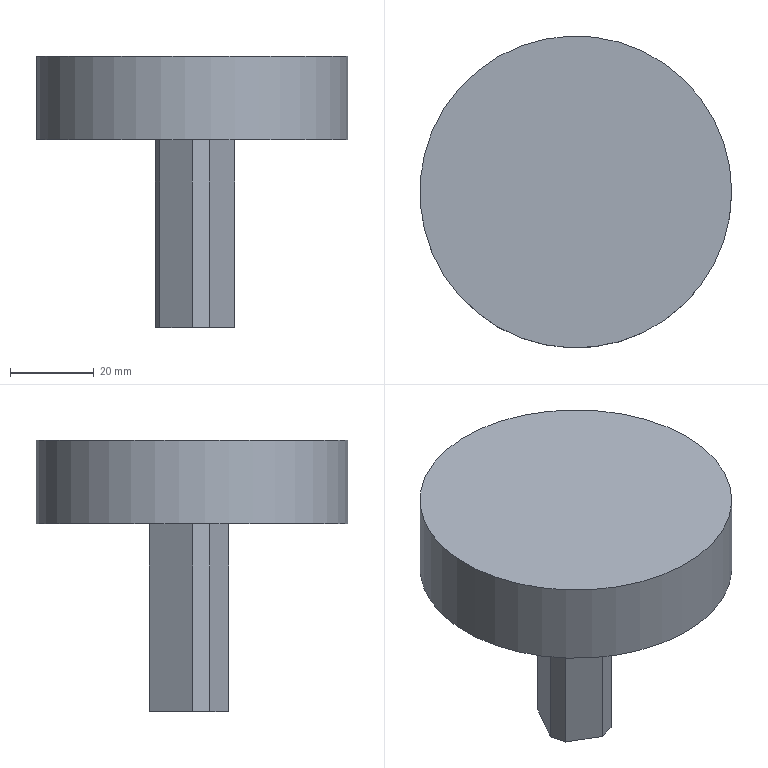Component | NX | CONNECTING_ROD | 1 solid | 17 faces | box 74.65 x 74.65 x 65 mm | volume 61981 mm3 | plane 12 | cylinder 4 | cone 1 | commonest cylinder face diameters 74.65 x1 66.65 x1 38.65 x1 8 x1
STEP:
#1=CARTESIAN_POINT('',(0.,0.,0.));
#2=DIRECTION('',(0.,0.,1.));
#3=DIRECTION('',(1.,0.,0.));
#4=AXIS2_PLACEMENT_3D('',#1,#2,#3);
#5=CARTESIAN_POINT('',(-5.912,-1.741,-7.5));
#6=VERTEX_POINT('',#5);
#7=CARTESIAN_POINT('',(3.75,14.995,-7.5));
#8=DIRECTION('',(0.,0.,-1.));
#9=DIRECTION('',(-0.5,-0.866,0.));
#10=AXIS2_PLACEMENT_3D('',#7,#8,#9);
#11=CIRCLE('',#10,19.325);
#12=CARTESIAN_POINT('',(3.75,14.995,-7.5));
#13=DIRECTION('',(0.,0.,-1.));
#14=DIRECTION('',(-0.5,-0.866,0.));
#15=AXIS2_PLACEMENT_3D('',#12,#13,#14);
#16=PLANE('',#15);
#17=CARTESIAN_POINT('',(0.,0.));
#18=DIRECTION('',(1.,0.));
#19=AXIS2_PLACEMENT_2D('',#17,#18);
#20=CIRCLE('',#19,19.325);
#21=(GEOMETRIC_REPRESENTATION_CONTEXT(2)PARAMETRIC_REPRESENTATION_CONTEXT()REPRESENTATION_CONTEXT('',''));
#22=DEFINITIONAL_REPRESENTATION('',(#20),#21);
#23=PCURVE('',#16,#22);
#24=CARTESIAN_POINT('',(3.75,14.995,7.5));
#25=DIRECTION('',(0.,0.,-1.));
#26=DIRECTION('',(-0.5,-0.866,0.));
#27=AXIS2_PLACEMENT_3D('',#24,#25,#26);
#28=CYLINDRICAL_SURFACE('',#27,19.325);
#29=CARTESIAN_POINT('',(0.,15.));
#30=DIRECTION('',(1.,0.));
#31=VECTOR('',#30,1.);
#32=LINE('',#29,#31);
#33=(GEOMETRIC_REPRESENTATION_CONTEXT(2)PARAMETRIC_REPRESENTATION_CONTEXT()REPRESENTATION_CONTEXT('',''));
#34=DEFINITIONAL_REPRESENTATION('',(#32),#33);
#35=PCURVE('',#28,#34);
#36=SURFACE_CURVE('',#11,(#23,#35),.PCURVE_S1.);
#37=EDGE_CURVE('',#6,#6,#36,.T.);
#38=ORIENTED_EDGE('',*,*,#37,.T.);
#39=EDGE_LOOP('',(#38));
#40=FACE_BOUND('',#39,.T.);
#41=CARTESIAN_POINT('',(1.005,25.24,-7.5));
#42=VERTEX_POINT('',#41);
#43=CARTESIAN_POINT('',(-4.995,14.848,-7.5));
#44=VERTEX_POINT('',#43);
#45=CARTESIAN_POINT('',(1.005,25.24,-7.5));
#46=DIRECTION('',(-0.5,-0.866,0.));
#47=VECTOR('',#46,1.);
#48=LINE('',#45,#47);
#49=CARTESIAN_POINT('',(-7.5,7.5));
#50=DIRECTION('',(1.,0.));
#51=VECTOR('',#50,1.);
#52=LINE('',#49,#51);
#53=(GEOMETRIC_REPRESENTATION_CONTEXT(2)PARAMETRIC_REPRESENTATION_CONTEXT()REPRESENTATION_CONTEXT('',''));
#54=DEFINITIONAL_REPRESENTATION('',(#52),#53);
#55=PCURVE('',#16,#54);
#56=CARTESIAN_POINT('',(1.005,25.24,-52.5));
#57=DIRECTION('',(-0.866,0.5,0.));
#58=DIRECTION('',(0.,0.,-1.));
#59=AXIS2_PLACEMENT_3D('',#56,#57,#58);
#60=PLANE('',#59);
#61=CARTESIAN_POINT('',(-45.,0.));
#62=DIRECTION('',(0.,1.));
#63=VECTOR('',#62,1.);
#64=LINE('',#61,#63);
#65=(GEOMETRIC_REPRESENTATION_CONTEXT(2)PARAMETRIC_REPRESENTATION_CONTEXT()REPRESENTATION_CONTEXT('',''));
#66=DEFINITIONAL_REPRESENTATION('',(#64),#65);
#67=PCURVE('',#60,#66);
#68=SURFACE_CURVE('',#48,(#55,#67),.PCURVE_S1.);
#69=EDGE_CURVE('',#42,#44,#68,.T.);
#70=ORIENTED_EDGE('',*,*,#69,.T.);
#71=CARTESIAN_POINT('',(-3.897,10.75,-7.5));
#72=VERTEX_POINT('',#71);
#73=CARTESIAN_POINT('',(-4.995,14.848,-7.5));
#74=DIRECTION('',(0.2588,-0.9659,0.));
#75=VECTOR('',#74,1.);
#76=LINE('',#73,#75);
#77=CARTESIAN_POINT('',(4.5,7.5));
#78=DIRECTION('',(0.7071,-0.7071));
#79=VECTOR('',#78,1.);
#80=LINE('',#77,#79);
#81=(GEOMETRIC_REPRESENTATION_CONTEXT(2)PARAMETRIC_REPRESENTATION_CONTEXT()REPRESENTATION_CONTEXT('',''));
#82=DEFINITIONAL_REPRESENTATION('',(#80),#81);
#83=PCURVE('',#16,#82);
#84=CARTESIAN_POINT('',(-4.995,14.848,-52.5));
#85=DIRECTION('',(0.9659,0.2588,0.));
#86=DIRECTION('',(0.,0.,1.));
#87=AXIS2_PLACEMENT_3D('',#84,#85,#86);
#88=PLANE('',#87);
#89=CARTESIAN_POINT('',(45.,0.));
#90=DIRECTION('',(0.,1.));
#91=VECTOR('',#90,1.);
#92=LINE('',#89,#91);
#93=(GEOMETRIC_REPRESENTATION_CONTEXT(2)PARAMETRIC_REPRESENTATION_CONTEXT()REPRESENTATION_CONTEXT('',''));
#94=DEFINITIONAL_REPRESENTATION('',(#92),#93);
#95=PCURVE('',#88,#94);
#96=SURFACE_CURVE('',#76,(#83,#95),.PCURVE_S1.);
#97=EDGE_CURVE('',#44,#72,#96,.T.);
#98=ORIENTED_EDGE('',*,*,#97,.T.);
#99=CARTESIAN_POINT('',(3.897,6.25,-7.5));
#100=VERTEX_POINT('',#99);
#101=CARTESIAN_POINT('',(-6.495,12.25,-7.5));
#102=DIRECTION('',(0.866,-0.5,0.));
#103=VECTOR('',#102,1.);
#104=LINE('',#101,#103);
#105=CARTESIAN_POINT('',(7.5,7.5));
#106=DIRECTION('',(0.,-1.));
#107=VECTOR('',#106,1.);
#108=LINE('',#105,#107);
#109=(GEOMETRIC_REPRESENTATION_CONTEXT(2)PARAMETRIC_REPRESENTATION_CONTEXT()REPRESENTATION_CONTEXT('',''));
#110=DEFINITIONAL_REPRESENTATION('',(#108),#109);
#111=PCURVE('',#16,#110);
#112=CARTESIAN_POINT('',(-6.495,12.25,-52.5));
#113=DIRECTION('',(-0.5,-0.866,0.));
#114=DIRECTION('',(0.,0.,1.));
#115=AXIS2_PLACEMENT_3D('',#112,#113,#114);
#116=PLANE('',#115);
#117=CARTESIAN_POINT('',(45.,0.));
#118=DIRECTION('',(0.,-1.));
#119=VECTOR('',#118,1.);
#120=LINE('',#117,#119);
#121=(GEOMETRIC_REPRESENTATION_CONTEXT(2)PARAMETRIC_REPRESENTATION_CONTEXT()REPRESENTATION_CONTEXT('',''));
#122=DEFINITIONAL_REPRESENTATION('',(#120),#121);
#123=PCURVE('',#116,#122);
#124=SURFACE_CURVE('',#104,(#111,#123),.PCURVE_S1.);
#125=EDGE_CURVE('',#72,#100,#124,.T.);
#126=ORIENTED_EDGE('',*,*,#125,.T.);
#127=CARTESIAN_POINT('',(7.995,7.348,-7.5));
#128=VERTEX_POINT('',#127);
#129=CARTESIAN_POINT('',(3.897,6.25,-7.5));
#130=DIRECTION('',(0.9659,0.2588,0.));
#131=VECTOR('',#130,1.);
#132=LINE('',#129,#131);
#133=CARTESIAN_POINT('',(7.5,-4.5));
#134=DIRECTION('',(-0.7071,-0.7071));
#135=VECTOR('',#134,1.);
#136=LINE('',#133,#135);
#137=(GEOMETRIC_REPRESENTATION_CONTEXT(2)PARAMETRIC_REPRESENTATION_CONTEXT()REPRESENTATION_CONTEXT('',''));
#138=DEFINITIONAL_REPRESENTATION('',(#136),#137);
#139=PCURVE('',#16,#138);
#140=CARTESIAN_POINT('',(3.897,6.25,-52.5));
#141=DIRECTION('',(-0.2588,0.9659,0.));
#142=DIRECTION('',(0.,0.,1.));
#143=AXIS2_PLACEMENT_3D('',#140,#141,#142);
#144=PLANE('',#143);
#145=CARTESIAN_POINT('',(45.,0.));
#146=DIRECTION('',(0.,1.));
#147=VECTOR('',#146,1.);
#148=LINE('',#145,#147);
#149=(GEOMETRIC_REPRESENTATION_CONTEXT(2)PARAMETRIC_REPRESENTATION_CONTEXT()REPRESENTATION_CONTEXT('',''));
#150=DEFINITIONAL_REPRESENTATION('',(#148),#149);
#151=PCURVE('',#144,#150);
#152=SURFACE_CURVE('',#132,(#139,#151),.PCURVE_S1.);
#153=EDGE_CURVE('',#100,#128,#152,.T.);
#154=ORIENTED_EDGE('',*,*,#153,.T.);
#155=CARTESIAN_POINT('',(13.995,17.74,-7.5));
#156=VERTEX_POINT('',#155);
#157=CARTESIAN_POINT('',(6.495,4.75,-7.5));
#158=DIRECTION('',(0.5,0.866,0.));
#159=VECTOR('',#158,1.);
#160=LINE('',#157,#159);
#161=CARTESIAN_POINT('',(7.5,-7.5));
#162=DIRECTION('',(-1.,0.));
#163=VECTOR('',#162,1.);
#164=LINE('',#161,#163);
#165=(GEOMETRIC_REPRESENTATION_CONTEXT(2)PARAMETRIC_REPRESENTATION_CONTEXT()REPRESENTATION_CONTEXT('',''));
#166=DEFINITIONAL_REPRESENTATION('',(#164),#165);
#167=PCURVE('',#16,#166);
#168=CARTESIAN_POINT('',(6.495,4.75,-52.5));
#169=DIRECTION('',(0.866,-0.5,0.));
#170=DIRECTION('',(0.,0.,1.));
#171=AXIS2_PLACEMENT_3D('',#168,#169,#170);
#172=PLANE('',#171);
#173=CARTESIAN_POINT('',(45.,0.));
#174=DIRECTION('',(0.,-1.));
#175=VECTOR('',#174,1.);
#176=LINE('',#173,#175);
#177=(GEOMETRIC_REPRESENTATION_CONTEXT(2)PARAMETRIC_REPRESENTATION_CONTEXT()REPRESENTATION_CONTEXT('',''));
#178=DEFINITIONAL_REPRESENTATION('',(#176),#177);
#179=PCURVE('',#172,#178);
#180=SURFACE_CURVE('',#160,(#167,#179),.PCURVE_S1.);
#181=EDGE_CURVE('',#128,#156,#180,.T.);
#182=ORIENTED_EDGE('',*,*,#181,.T.);
#183=CARTESIAN_POINT('',(13.995,17.74,-7.5));
#184=DIRECTION('',(-0.866,0.5,0.));
#185=VECTOR('',#184,1.);
#186=LINE('',#183,#185);
#187=CARTESIAN_POINT('',(-7.5,-7.5));
#188=DIRECTION('',(0.,1.));
#189=VECTOR('',#188,1.);
#190=LINE('',#187,#189);
#191=(GEOMETRIC_REPRESENTATION_CONTEXT(2)PARAMETRIC_REPRESENTATION_CONTEXT()REPRESENTATION_CONTEXT('',''));
#192=DEFINITIONAL_REPRESENTATION('',(#190),#191);
#193=PCURVE('',#16,#192);
#194=CARTESIAN_POINT('',(13.995,17.74,-52.5));
#195=DIRECTION('',(0.5,0.866,0.));
#196=DIRECTION('',(0.,0.,-1.));
#197=AXIS2_PLACEMENT_3D('',#194,#195,#196);
#198=PLANE('',#197);
#199=CARTESIAN_POINT('',(-45.,0.));
#200=DIRECTION('',(0.,1.));
#201=VECTOR('',#200,1.);
#202=LINE('',#199,#201);
#203=(GEOMETRIC_REPRESENTATION_CONTEXT(2)PARAMETRIC_REPRESENTATION_CONTEXT()REPRESENTATION_CONTEXT('',''));
#204=DEFINITIONAL_REPRESENTATION('',(#202),#203);
#205=PCURVE('',#198,#204);
#206=SURFACE_CURVE('',#186,(#193,#205),.PCURVE_S1.);
#207=EDGE_CURVE('',#156,#42,#206,.T.);
#208=ORIENTED_EDGE('',*,*,#207,.T.);
#209=EDGE_LOOP('',(#70,#98,#126,#154,#182,#208));
#210=FACE_BOUND('',#209,.T.);
#211=ADVANCED_FACE('',(#40,#210),#16,.T.);
#212=CARTESIAN_POINT('',(-12.912,-13.865,-7.5));
#213=VERTEX_POINT('',#212);
#214=CARTESIAN_POINT('',(3.75,14.995,-7.5));
#215=DIRECTION('',(0.,0.,-1.));
#216=DIRECTION('',(-0.5,-0.866,0.));
#217=AXIS2_PLACEMENT_3D('',#214,#215,#216);
#218=CIRCLE('',#217,33.325);
#219=CARTESIAN_POINT('',(3.75,14.995,-7.5));
#220=DIRECTION('',(0.,0.,-1.));
#221=DIRECTION('',(-0.5,-0.866,0.));
#222=AXIS2_PLACEMENT_3D('',#219,#220,#221);
#223=PLANE('',#222);
#224=CARTESIAN_POINT('',(0.,0.));
#225=DIRECTION('',(1.,0.));
#226=AXIS2_PLACEMENT_2D('',#224,#225);
#227=CIRCLE('',#226,33.325);
#228=(GEOMETRIC_REPRESENTATION_CONTEXT(2)PARAMETRIC_REPRESENTATION_CONTEXT()REPRESENTATION_CONTEXT('',''));
#229=DEFINITIONAL_REPRESENTATION('',(#227),#228);
#230=PCURVE('',#223,#229);
#231=CARTESIAN_POINT('',(3.75,14.995,7.5));
#232=DIRECTION('',(0.,0.,-1.));
#233=DIRECTION('',(-0.5,-0.866,0.));
#234=AXIS2_PLACEMENT_3D('',#231,#232,#233);
#235=CYLINDRICAL_SURFACE('',#234,33.325);
#236=CARTESIAN_POINT('',(0.,15.));
#237=DIRECTION('',(1.,0.));
#238=VECTOR('',#237,1.);
#239=LINE('',#236,#238);
#240=(GEOMETRIC_REPRESENTATION_CONTEXT(2)PARAMETRIC_REPRESENTATION_CONTEXT()REPRESENTATION_CONTEXT('',''));
#241=DEFINITIONAL_REPRESENTATION('',(#239),#240);
#242=PCURVE('',#235,#241);
#243=SURFACE_CURVE('',#218,(#230,#242),.PCURVE_S1.);
#244=EDGE_CURVE('',#213,#213,#243,.T.);
#245=ORIENTED_EDGE('',*,*,#244,.F.);
#246=EDGE_LOOP('',(#245));
#247=FACE_BOUND('',#246,.T.);
#248=CARTESIAN_POINT('',(-14.912,-17.329,-7.5));
#249=VERTEX_POINT('',#248);
#250=CARTESIAN_POINT('',(3.75,14.995,-7.5));
#251=DIRECTION('',(0.,0.,1.));
#252=DIRECTION('',(-0.5,-0.866,0.));
#253=AXIS2_PLACEMENT_3D('',#250,#251,#252);
#254=CIRCLE('',#253,37.325);
#255=CARTESIAN_POINT('',(37.325,0.));
#256=CARTESIAN_POINT('',(37.325,-64.649));
#257=CARTESIAN_POINT('',(-18.663,-32.324));
#258=CARTESIAN_POINT('',(-74.65,-0.));
#259=CARTESIAN_POINT('',(-18.663,32.324));
#260=CARTESIAN_POINT('',(37.325,64.649));
#261=CARTESIAN_POINT('',(37.325,0.));
#262=(BOUNDED_CURVE()B_SPLINE_CURVE(2,(#255,#256,#257,#258,#259,#260,#261),.UNSPECIFIED.,.T.,.F.)B_SPLINE_CURVE_WITH_KNOTS((1,2,2,2,2,1),(-2.094,0.,2.094,4.189,6.283,8.378),.UNSPECIFIED.)CURVE()GEOMETRIC_REPRESENTATION_ITEM()RATIONAL_B_SPLINE_CURVE((1.,0.5,1.,0.5,1.,0.5,1.))REPRESENTATION_ITEM(''));
#263=(GEOMETRIC_REPRESENTATION_CONTEXT(2)PARAMETRIC_REPRESENTATION_CONTEXT()REPRESENTATION_CONTEXT('',''));
#264=DEFINITIONAL_REPRESENTATION('',(#262),#263);
#265=PCURVE('',#223,#264);
#266=CARTESIAN_POINT('',(3.75,14.995,12.5));
#267=DIRECTION('',(0.,0.,-1.));
#268=DIRECTION('',(-0.5,-0.866,0.));
#269=AXIS2_PLACEMENT_3D('',#266,#267,#268);
#270=CYLINDRICAL_SURFACE('',#269,37.325);
#271=CARTESIAN_POINT('',(6.283,20.));
#272=DIRECTION('',(-1.,0.));
#273=VECTOR('',#272,1.);
#274=LINE('',#271,#273);
#275=(GEOMETRIC_REPRESENTATION_CONTEXT(2)PARAMETRIC_REPRESENTATION_CONTEXT()REPRESENTATION_CONTEXT('',''));
#276=DEFINITIONAL_REPRESENTATION('',(#274),#275);
#277=PCURVE('',#270,#276);
#278=SURFACE_CURVE('',#254,(#265,#277),.PCURVE_S1.);
#279=EDGE_CURVE('',#249,#249,#278,.T.);
#280=ORIENTED_EDGE('',*,*,#279,.F.);
#281=EDGE_LOOP('',(#280));
#282=FACE_BOUND('',#281,.T.);
#283=ADVANCED_FACE('',(#247,#282),#223,.T.);
#284=CARTESIAN_POINT('',(-14.912,-17.329,12.5));
#285=VERTEX_POINT('',#284);
#286=CARTESIAN_POINT('',(3.75,14.995,12.5));
#287=DIRECTION('',(0.,0.,-1.));
#288=DIRECTION('',(-0.5,-0.866,0.));
#289=AXIS2_PLACEMENT_3D('',#286,#287,#288);
#290=CIRCLE('',#289,37.325);
#291=CARTESIAN_POINT('',(3.75,14.995,12.5));
#292=DIRECTION('',(0.,0.,1.));
#293=DIRECTION('',(0.5,0.866,0.));
#294=AXIS2_PLACEMENT_3D('',#291,#292,#293);
#295=PLANE('',#294);
#296=CARTESIAN_POINT('',(-37.325,0.));
#297=CARTESIAN_POINT('',(-37.325,64.649));
#298=CARTESIAN_POINT('',(18.663,32.324));
#299=CARTESIAN_POINT('',(74.65,0.));
#300=CARTESIAN_POINT('',(18.663,-32.324));
#301=CARTESIAN_POINT('',(-37.325,-64.649));
#302=CARTESIAN_POINT('',(-37.325,0.));
#303=(BOUNDED_CURVE()B_SPLINE_CURVE(2,(#296,#297,#298,#299,#300,#301,#302),.UNSPECIFIED.,.T.,.F.)B_SPLINE_CURVE_WITH_KNOTS((1,2,2,2,2,1),(-2.094,0.,2.094,4.189,6.283,8.378),.UNSPECIFIED.)CURVE()GEOMETRIC_REPRESENTATION_ITEM()RATIONAL_B_SPLINE_CURVE((1.,0.5,1.,0.5,1.,0.5,1.))REPRESENTATION_ITEM(''));
#304=(GEOMETRIC_REPRESENTATION_CONTEXT(2)PARAMETRIC_REPRESENTATION_CONTEXT()REPRESENTATION_CONTEXT('',''));
#305=DEFINITIONAL_REPRESENTATION('',(#303),#304);
#306=PCURVE('',#295,#305);
#307=CARTESIAN_POINT('',(0.,0.));
#308=DIRECTION('',(1.,0.));
#309=VECTOR('',#308,1.);
#310=LINE('',#307,#309);
#311=(GEOMETRIC_REPRESENTATION_CONTEXT(2)PARAMETRIC_REPRESENTATION_CONTEXT()REPRESENTATION_CONTEXT('',''));
#312=DEFINITIONAL_REPRESENTATION('',(#310),#311);
#313=PCURVE('',#270,#312);
#314=SURFACE_CURVE('',#290,(#306,#313),.PCURVE_S1.);
#315=EDGE_CURVE('',#285,#285,#314,.T.);
#316=ORIENTED_EDGE('',*,*,#315,.F.);
#317=EDGE_LOOP('',(#316));
#318=FACE_BOUND('',#317,.T.);
#319=ADVANCED_FACE('',(#318),#295,.T.);
#320=ORIENTED_EDGE('',*,*,#279,.T.);
#321=CARTESIAN_POINT('',(-14.912,-17.329,12.5));
#322=CARTESIAN_POINT('',(-14.912,-17.329,-7.5));
#323=B_SPLINE_CURVE_WITH_KNOTS('',1,(#321,#322),.UNSPECIFIED.,.F.,.F.,(2,2),(0.,20.),.PIECEWISE_BEZIER_KNOTS.);
#324=CARTESIAN_POINT('',(0.,0.));
#325=DIRECTION('',(0.,1.));
#326=VECTOR('',#325,1.);
#327=LINE('',#324,#326);
#328=(GEOMETRIC_REPRESENTATION_CONTEXT(2)PARAMETRIC_REPRESENTATION_CONTEXT()REPRESENTATION_CONTEXT('',''));
#329=DEFINITIONAL_REPRESENTATION('',(#327),#328);
#330=PCURVE('',#270,#329);
#331=CARTESIAN_POINT('',(6.283,0.));
#332=DIRECTION('',(0.,1.));
#333=VECTOR('',#332,1.);
#334=LINE('',#331,#333);
#335=(GEOMETRIC_REPRESENTATION_CONTEXT(2)PARAMETRIC_REPRESENTATION_CONTEXT()REPRESENTATION_CONTEXT('',''));
#336=DEFINITIONAL_REPRESENTATION('',(#334),#335);
#337=PCURVE('',#270,#336);
#338=SEAM_CURVE('',#323,(#330,#337),.PCURVE_S1.);
#339=EDGE_CURVE('',#285,#249,#338,.T.);
#340=ORIENTED_EDGE('',*,*,#339,.F.);
#341=ORIENTED_EDGE('',*,*,#315,.T.);
#342=ORIENTED_EDGE('',*,*,#339,.T.);
#343=EDGE_LOOP('',(#320,#340,#341,#342));
#344=FACE_BOUND('',#343,.T.);
#345=ADVANCED_FACE('',(#344),#270,.T.);
#346=CARTESIAN_POINT('',(-12.912,-13.865,7.5));
#347=VERTEX_POINT('',#346);
#348=CARTESIAN_POINT('',(3.75,14.995,7.5));
#349=DIRECTION('',(0.,0.,1.));
#350=DIRECTION('',(-0.5,-0.866,0.));
#351=AXIS2_PLACEMENT_3D('',#348,#349,#350);
#352=CIRCLE('',#351,33.325);
#353=CARTESIAN_POINT('',(6.283,0.));
#354=DIRECTION('',(-1.,0.));
#355=VECTOR('',#354,1.);
#356=LINE('',#353,#355);
#357=(GEOMETRIC_REPRESENTATION_CONTEXT(2)PARAMETRIC_REPRESENTATION_CONTEXT()REPRESENTATION_CONTEXT('',''));
#358=DEFINITIONAL_REPRESENTATION('',(#356),#357);
#359=PCURVE('',#235,#358);
#360=CARTESIAN_POINT('',(3.75,14.995,7.5));
#361=DIRECTION('',(0.,0.,-1.));
#362=DIRECTION('',(-0.5,-0.866,0.));
#363=AXIS2_PLACEMENT_3D('',#360,#361,#362);
#364=PLANE('',#363);
#365=CARTESIAN_POINT('',(33.325,0.));
#366=CARTESIAN_POINT('',(33.325,-57.721));
#367=CARTESIAN_POINT('',(-16.663,-28.86));
#368=CARTESIAN_POINT('',(-66.65,-0.));
#369=CARTESIAN_POINT('',(-16.663,28.86));
#370=CARTESIAN_POINT('',(33.325,57.721));
#371=CARTESIAN_POINT('',(33.325,0.));
#372=(BOUNDED_CURVE()B_SPLINE_CURVE(2,(#365,#366,#367,#368,#369,#370,#371),.UNSPECIFIED.,.T.,.F.)B_SPLINE_CURVE_WITH_KNOTS((1,2,2,2,2,1),(-2.094,0.,2.094,4.189,6.283,8.378),.UNSPECIFIED.)CURVE()GEOMETRIC_REPRESENTATION_ITEM()RATIONAL_B_SPLINE_CURVE((1.,0.5,1.,0.5,1.,0.5,1.))REPRESENTATION_ITEM(''));
#373=(GEOMETRIC_REPRESENTATION_CONTEXT(2)PARAMETRIC_REPRESENTATION_CONTEXT()REPRESENTATION_CONTEXT('',''));
#374=DEFINITIONAL_REPRESENTATION('',(#372),#373);
#375=PCURVE('',#364,#374);
#376=SURFACE_CURVE('',#352,(#359,#375),.PCURVE_S1.);
#377=EDGE_CURVE('',#347,#347,#376,.T.);
#378=ORIENTED_EDGE('',*,*,#377,.F.);
#379=CARTESIAN_POINT('',(-12.912,-13.865,7.5));
#380=CARTESIAN_POINT('',(-12.912,-13.865,-7.5));
#381=B_SPLINE_CURVE_WITH_KNOTS('',1,(#379,#380),.UNSPECIFIED.,.F.,.F.,(2,2),(0.,15.),.PIECEWISE_BEZIER_KNOTS.);
#382=CARTESIAN_POINT('',(6.283,0.));
#383=DIRECTION('',(0.,1.));
#384=VECTOR('',#383,1.);
#385=LINE('',#382,#384);
#386=(GEOMETRIC_REPRESENTATION_CONTEXT(2)PARAMETRIC_REPRESENTATION_CONTEXT()REPRESENTATION_CONTEXT('',''));
#387=DEFINITIONAL_REPRESENTATION('',(#385),#386);
#388=PCURVE('',#235,#387);
#389=CARTESIAN_POINT('',(0.,0.));
#390=DIRECTION('',(0.,1.));
#391=VECTOR('',#390,1.);
#392=LINE('',#389,#391);
#393=(GEOMETRIC_REPRESENTATION_CONTEXT(2)PARAMETRIC_REPRESENTATION_CONTEXT()REPRESENTATION_CONTEXT('',''));
#394=DEFINITIONAL_REPRESENTATION('',(#392),#393);
#395=PCURVE('',#235,#394);
#396=SEAM_CURVE('',#381,(#388,#395),.PCURVE_S1.);
#397=EDGE_CURVE('',#347,#213,#396,.T.);
#398=ORIENTED_EDGE('',*,*,#397,.T.);
#399=ORIENTED_EDGE('',*,*,#244,.F.);
#400=ORIENTED_EDGE('',*,*,#397,.F.);
#401=EDGE_LOOP('',(#378,#398,#399,#400));
#402=FACE_BOUND('',#401,.F.);
#403=ADVANCED_FACE('',(#402),#235,.F.);
#404=CARTESIAN_POINT('',(-5.912,-1.741,7.5));
#405=VERTEX_POINT('',#404);
#406=CARTESIAN_POINT('',(3.75,14.995,7.5));
#407=DIRECTION('',(0.,0.,1.));
#408=DIRECTION('',(-0.5,-0.866,0.));
#409=AXIS2_PLACEMENT_3D('',#406,#407,#408);
#410=CIRCLE('',#409,19.325);
#411=CARTESIAN_POINT('',(6.283,0.));
#412=DIRECTION('',(-1.,0.));
#413=VECTOR('',#412,1.);
#414=LINE('',#411,#413);
#415=(GEOMETRIC_REPRESENTATION_CONTEXT(2)PARAMETRIC_REPRESENTATION_CONTEXT()REPRESENTATION_CONTEXT('',''));
#416=DEFINITIONAL_REPRESENTATION('',(#414),#415);
#417=PCURVE('',#28,#416);
#418=CARTESIAN_POINT('',(19.325,0.));
#419=CARTESIAN_POINT('',(19.325,-33.472));
#420=CARTESIAN_POINT('',(-9.662,-16.736));
#421=CARTESIAN_POINT('',(-38.65,-0.));
#422=CARTESIAN_POINT('',(-9.662,16.736));
#423=CARTESIAN_POINT('',(19.325,33.472));
#424=CARTESIAN_POINT('',(19.325,0.));
#425=(BOUNDED_CURVE()B_SPLINE_CURVE(2,(#418,#419,#420,#421,#422,#423,#424),.UNSPECIFIED.,.T.,.F.)B_SPLINE_CURVE_WITH_KNOTS((1,2,2,2,2,1),(-2.094,0.,2.094,4.189,6.283,8.378),.UNSPECIFIED.)CURVE()GEOMETRIC_REPRESENTATION_ITEM()RATIONAL_B_SPLINE_CURVE((1.,0.5,1.,0.5,1.,0.5,1.))REPRESENTATION_ITEM(''));
#426=(GEOMETRIC_REPRESENTATION_CONTEXT(2)PARAMETRIC_REPRESENTATION_CONTEXT()REPRESENTATION_CONTEXT('',''));
#427=DEFINITIONAL_REPRESENTATION('',(#425),#426);
#428=PCURVE('',#364,#427);
#429=SURFACE_CURVE('',#410,(#417,#428),.PCURVE_S1.);
#430=EDGE_CURVE('',#405,#405,#429,.T.);
#431=ORIENTED_EDGE('',*,*,#430,.F.);
#432=CARTESIAN_POINT('',(-5.912,-1.741,7.5));
#433=CARTESIAN_POINT('',(-5.912,-1.741,-7.5));
#434=B_SPLINE_CURVE_WITH_KNOTS('',1,(#432,#433),.UNSPECIFIED.,.F.,.F.,(2,2),(0.,15.),.PIECEWISE_BEZIER_KNOTS.);
#435=CARTESIAN_POINT('',(6.283,0.));
#436=DIRECTION('',(0.,1.));
#437=VECTOR('',#436,1.);
#438=LINE('',#435,#437);
#439=(GEOMETRIC_REPRESENTATION_CONTEXT(2)PARAMETRIC_REPRESENTATION_CONTEXT()REPRESENTATION_CONTEXT('',''));
#440=DEFINITIONAL_REPRESENTATION('',(#438),#439);
#441=PCURVE('',#28,#440);
#442=CARTESIAN_POINT('',(0.,0.));
#443=DIRECTION('',(0.,1.));
#444=VECTOR('',#443,1.);
#445=LINE('',#442,#444);
#446=(GEOMETRIC_REPRESENTATION_CONTEXT(2)PARAMETRIC_REPRESENTATION_CONTEXT()REPRESENTATION_CONTEXT('',''));
#447=DEFINITIONAL_REPRESENTATION('',(#445),#446);
#448=PCURVE('',#28,#447);
#449=SEAM_CURVE('',#434,(#441,#448),.PCURVE_S1.);
#450=EDGE_CURVE('',#405,#6,#449,.T.);
#451=ORIENTED_EDGE('',*,*,#450,.T.);
#452=ORIENTED_EDGE('',*,*,#37,.F.);
#453=ORIENTED_EDGE('',*,*,#450,.F.);
#454=EDGE_LOOP('',(#431,#451,#452,#453));
#455=FACE_BOUND('',#454,.T.);
#456=ADVANCED_FACE('',(#455),#28,.T.);
#457=ORIENTED_EDGE('',*,*,#377,.F.);
#458=EDGE_LOOP('',(#457));
#459=FACE_BOUND('',#458,.T.);
#460=ORIENTED_EDGE('',*,*,#430,.T.);
#461=EDGE_LOOP('',(#460));
#462=FACE_BOUND('',#461,.T.);
#463=ADVANCED_FACE('',(#459,#462),#364,.T.);
#464=ORIENTED_EDGE('',*,*,#125,.F.);
#465=CARTESIAN_POINT('',(-3.897,10.75,-52.5));
#466=VERTEX_POINT('',#465);
#467=CARTESIAN_POINT('',(-3.897,10.75,-52.5));
#468=DIRECTION('',(0.,0.,-1.));
#469=VECTOR('',#468,1.);
#470=LINE('',#467,#469);
#471=CARTESIAN_POINT('',(0.,-3.));
#472=DIRECTION('',(-1.,0.));
#473=VECTOR('',#472,1.);
#474=LINE('',#471,#473);
#475=(GEOMETRIC_REPRESENTATION_CONTEXT(2)PARAMETRIC_REPRESENTATION_CONTEXT()REPRESENTATION_CONTEXT('',''));
#476=DEFINITIONAL_REPRESENTATION('',(#474),#475);
#477=PCURVE('',#116,#476);
#478=CARTESIAN_POINT('',(0.,4.243));
#479=DIRECTION('',(-1.,0.));
#480=VECTOR('',#479,1.);
#481=LINE('',#478,#480);
#482=(GEOMETRIC_REPRESENTATION_CONTEXT(2)PARAMETRIC_REPRESENTATION_CONTEXT()REPRESENTATION_CONTEXT('',''));
#483=DEFINITIONAL_REPRESENTATION('',(#481),#482);
#484=PCURVE('',#88,#483);
#485=SURFACE_CURVE('',#470,(#477,#484),.PCURVE_S1.);
#486=EDGE_CURVE('',#72,#466,#485,.T.);
#487=ORIENTED_EDGE('',*,*,#486,.T.);
#488=CARTESIAN_POINT('',(3.897,6.25,-52.5));
#489=VERTEX_POINT('',#488);
#490=CARTESIAN_POINT('',(-6.495,12.25,-52.5));
#491=DIRECTION('',(0.866,-0.5,0.));
#492=VECTOR('',#491,1.);
#493=LINE('',#490,#492);
#494=CARTESIAN_POINT('',(0.,0.));
#495=DIRECTION('',(0.,-1.));
#496=VECTOR('',#495,1.);
#497=LINE('',#494,#496);
#498=(GEOMETRIC_REPRESENTATION_CONTEXT(2)PARAMETRIC_REPRESENTATION_CONTEXT()REPRESENTATION_CONTEXT('',''));
#499=DEFINITIONAL_REPRESENTATION('',(#497),#498);
#500=PCURVE('',#116,#499);
#501=CARTESIAN_POINT('',(3.75,14.995,-52.5));
#502=DIRECTION('',(0.,0.,1.));
#503=DIRECTION('',(0.5,0.866,0.));
#504=AXIS2_PLACEMENT_3D('',#501,#502,#503);
#505=PLANE('',#504);
#506=CARTESIAN_POINT('',(-7.5,7.5));
#507=DIRECTION('',(0.,-1.));
#508=VECTOR('',#507,1.);
#509=LINE('',#506,#508);
#510=(GEOMETRIC_REPRESENTATION_CONTEXT(2)PARAMETRIC_REPRESENTATION_CONTEXT()REPRESENTATION_CONTEXT('',''));
#511=DEFINITIONAL_REPRESENTATION('',(#509),#510);
#512=PCURVE('',#505,#511);
#513=SURFACE_CURVE('',#493,(#500,#512),.PCURVE_S1.);
#514=EDGE_CURVE('',#466,#489,#513,.T.);
#515=ORIENTED_EDGE('',*,*,#514,.T.);
#516=CARTESIAN_POINT('',(3.897,6.25,-52.5));
#517=DIRECTION('',(0.,0.,1.));
#518=VECTOR('',#517,1.);
#519=LINE('',#516,#518);
#520=CARTESIAN_POINT('',(0.,-12.));
#521=DIRECTION('',(1.,0.));
#522=VECTOR('',#521,1.);
#523=LINE('',#520,#522);
#524=(GEOMETRIC_REPRESENTATION_CONTEXT(2)PARAMETRIC_REPRESENTATION_CONTEXT()REPRESENTATION_CONTEXT('',''));
#525=DEFINITIONAL_REPRESENTATION('',(#523),#524);
#526=PCURVE('',#116,#525);
#527=CARTESIAN_POINT('',(0.,0.));
#528=DIRECTION('',(1.,0.));
#529=VECTOR('',#528,1.);
#530=LINE('',#527,#529);
#531=(GEOMETRIC_REPRESENTATION_CONTEXT(2)PARAMETRIC_REPRESENTATION_CONTEXT()REPRESENTATION_CONTEXT('',''));
#532=DEFINITIONAL_REPRESENTATION('',(#530),#531);
#533=PCURVE('',#144,#532);
#534=SURFACE_CURVE('',#519,(#526,#533),.PCURVE_S1.);
#535=EDGE_CURVE('',#489,#100,#534,.T.);
#536=ORIENTED_EDGE('',*,*,#535,.T.);
#537=EDGE_LOOP('',(#464,#487,#515,#536));
#538=FACE_BOUND('',#537,.T.);
#539=ADVANCED_FACE('',(#538),#116,.T.);
#540=ORIENTED_EDGE('',*,*,#181,.F.);
#541=CARTESIAN_POINT('',(7.995,7.348,-52.5));
#542=VERTEX_POINT('',#541);
#543=CARTESIAN_POINT('',(7.995,7.348,-52.5));
#544=DIRECTION('',(0.,0.,-1.));
#545=VECTOR('',#544,1.);
#546=LINE('',#543,#545);
#547=CARTESIAN_POINT('',(0.,-3.));
#548=DIRECTION('',(-1.,0.));
#549=VECTOR('',#548,1.);
#550=LINE('',#547,#549);
#551=(GEOMETRIC_REPRESENTATION_CONTEXT(2)PARAMETRIC_REPRESENTATION_CONTEXT()REPRESENTATION_CONTEXT('',''));
#552=DEFINITIONAL_REPRESENTATION('',(#550),#551);
#553=PCURVE('',#172,#552);
#554=CARTESIAN_POINT('',(0.,4.243));
#555=DIRECTION('',(-1.,0.));
#556=VECTOR('',#555,1.);
#557=LINE('',#554,#556);
#558=(GEOMETRIC_REPRESENTATION_CONTEXT(2)PARAMETRIC_REPRESENTATION_CONTEXT()REPRESENTATION_CONTEXT('',''));
#559=DEFINITIONAL_REPRESENTATION('',(#557),#558);
#560=PCURVE('',#144,#559);
#561=SURFACE_CURVE('',#546,(#553,#560),.PCURVE_S1.);
#562=EDGE_CURVE('',#128,#542,#561,.T.);
#563=ORIENTED_EDGE('',*,*,#562,.T.);
#564=CARTESIAN_POINT('',(13.995,17.74,-52.5));
#565=VERTEX_POINT('',#564);
#566=CARTESIAN_POINT('',(6.495,4.75,-52.5));
#567=DIRECTION('',(0.5,0.866,0.));
#568=VECTOR('',#567,1.);
#569=LINE('',#566,#568);
#570=CARTESIAN_POINT('',(0.,0.));
#571=DIRECTION('',(0.,-1.));
#572=VECTOR('',#571,1.);
#573=LINE('',#570,#572);
#574=(GEOMETRIC_REPRESENTATION_CONTEXT(2)PARAMETRIC_REPRESENTATION_CONTEXT()REPRESENTATION_CONTEXT('',''));
#575=DEFINITIONAL_REPRESENTATION('',(#573),#574);
#576=PCURVE('',#172,#575);
#577=CARTESIAN_POINT('',(-7.5,-7.5));
#578=DIRECTION('',(1.,0.));
#579=VECTOR('',#578,1.);
#580=LINE('',#577,#579);
#581=(GEOMETRIC_REPRESENTATION_CONTEXT(2)PARAMETRIC_REPRESENTATION_CONTEXT()REPRESENTATION_CONTEXT('',''));
#582=DEFINITIONAL_REPRESENTATION('',(#580),#581);
#583=PCURVE('',#505,#582);
#584=SURFACE_CURVE('',#569,(#576,#583),.PCURVE_S1.);
#585=EDGE_CURVE('',#542,#565,#584,.T.);
#586=ORIENTED_EDGE('',*,*,#585,.T.);
#587=CARTESIAN_POINT('',(13.995,17.74,-52.5));
#588=DIRECTION('',(0.,0.,1.));
#589=VECTOR('',#588,1.);
#590=LINE('',#587,#589);
#591=CARTESIAN_POINT('',(0.,-15.));
#592=DIRECTION('',(1.,0.));
#593=VECTOR('',#592,1.);
#594=LINE('',#591,#593);
#595=(GEOMETRIC_REPRESENTATION_CONTEXT(2)PARAMETRIC_REPRESENTATION_CONTEXT()REPRESENTATION_CONTEXT('',''));
#596=DEFINITIONAL_REPRESENTATION('',(#594),#595);
#597=PCURVE('',#172,#596);
#598=CARTESIAN_POINT('',(0.,0.));
#599=DIRECTION('',(-1.,0.));
#600=VECTOR('',#599,1.);
#601=LINE('',#598,#600);
#602=(GEOMETRIC_REPRESENTATION_CONTEXT(2)PARAMETRIC_REPRESENTATION_CONTEXT()REPRESENTATION_CONTEXT('',''));
#603=DEFINITIONAL_REPRESENTATION('',(#601),#602);
#604=PCURVE('',#198,#603);
#605=SURFACE_CURVE('',#590,(#597,#604),.PCURVE_S1.);
#606=EDGE_CURVE('',#565,#156,#605,.T.);
#607=ORIENTED_EDGE('',*,*,#606,.T.);
#608=EDGE_LOOP('',(#540,#563,#586,#607));
#609=FACE_BOUND('',#608,.T.);
#610=ADVANCED_FACE('',(#609),#172,.T.);
#611=ORIENTED_EDGE('',*,*,#207,.F.);
#612=ORIENTED_EDGE('',*,*,#606,.F.);
#613=CARTESIAN_POINT('',(1.005,25.24,-52.5));
#614=VERTEX_POINT('',#613);
#615=CARTESIAN_POINT('',(13.995,17.74,-52.5));
#616=DIRECTION('',(-0.866,0.5,0.));
#617=VECTOR('',#616,1.);
#618=LINE('',#615,#617);
#619=CARTESIAN_POINT('',(0.,0.));
#620=DIRECTION('',(0.,1.));
#621=VECTOR('',#620,1.);
#622=LINE('',#619,#621);
#623=(GEOMETRIC_REPRESENTATION_CONTEXT(2)PARAMETRIC_REPRESENTATION_CONTEXT()REPRESENTATION_CONTEXT('',''));
#624=DEFINITIONAL_REPRESENTATION('',(#622),#623);
#625=PCURVE('',#198,#624);
#626=CARTESIAN_POINT('',(7.5,-7.5));
#627=DIRECTION('',(0.,1.));
#628=VECTOR('',#627,1.);
#629=LINE('',#626,#628);
#630=(GEOMETRIC_REPRESENTATION_CONTEXT(2)PARAMETRIC_REPRESENTATION_CONTEXT()REPRESENTATION_CONTEXT('',''));
#631=DEFINITIONAL_REPRESENTATION('',(#629),#630);
#632=PCURVE('',#505,#631);
#633=SURFACE_CURVE('',#618,(#625,#632),.PCURVE_S1.);
#634=EDGE_CURVE('',#565,#614,#633,.T.);
#635=ORIENTED_EDGE('',*,*,#634,.T.);
#636=CARTESIAN_POINT('',(1.005,25.24,-52.5));
#637=DIRECTION('',(0.,0.,1.));
#638=VECTOR('',#637,1.);
#639=LINE('',#636,#638);
#640=CARTESIAN_POINT('',(0.,15.));
#641=DIRECTION('',(-1.,0.));
#642=VECTOR('',#641,1.);
#643=LINE('',#640,#642);
#644=(GEOMETRIC_REPRESENTATION_CONTEXT(2)PARAMETRIC_REPRESENTATION_CONTEXT()REPRESENTATION_CONTEXT('',''));
#645=DEFINITIONAL_REPRESENTATION('',(#643),#644);
#646=PCURVE('',#198,#645);
#647=CARTESIAN_POINT('',(0.,0.));
#648=DIRECTION('',(-1.,0.));
#649=VECTOR('',#648,1.);
#650=LINE('',#647,#649);
#651=(GEOMETRIC_REPRESENTATION_CONTEXT(2)PARAMETRIC_REPRESENTATION_CONTEXT()REPRESENTATION_CONTEXT('',''));
#652=DEFINITIONAL_REPRESENTATION('',(#650),#651);
#653=PCURVE('',#60,#652);
#654=SURFACE_CURVE('',#639,(#646,#653),.PCURVE_S1.);
#655=EDGE_CURVE('',#614,#42,#654,.T.);
#656=ORIENTED_EDGE('',*,*,#655,.T.);
#657=EDGE_LOOP('',(#611,#612,#635,#656));
#658=FACE_BOUND('',#657,.T.);
#659=ADVANCED_FACE('',(#658),#198,.T.);
#660=CARTESIAN_POINT('',(-4.995,14.848,-52.5));
#661=VERTEX_POINT('',#660);
#662=CARTESIAN_POINT('',(1.005,25.24,-52.5));
#663=DIRECTION('',(-0.5,-0.866,0.));
#664=VECTOR('',#663,1.);
#665=LINE('',#662,#664);
#666=CARTESIAN_POINT('',(0.,0.));
#667=DIRECTION('',(0.,1.));
#668=VECTOR('',#667,1.);
#669=LINE('',#666,#668);
#670=(GEOMETRIC_REPRESENTATION_CONTEXT(2)PARAMETRIC_REPRESENTATION_CONTEXT()REPRESENTATION_CONTEXT('',''));
#671=DEFINITIONAL_REPRESENTATION('',(#669),#670);
#672=PCURVE('',#60,#671);
#673=CARTESIAN_POINT('',(7.5,7.5));
#674=DIRECTION('',(-1.,0.));
#675=VECTOR('',#674,1.);
#676=LINE('',#673,#675);
#677=(GEOMETRIC_REPRESENTATION_CONTEXT(2)PARAMETRIC_REPRESENTATION_CONTEXT()REPRESENTATION_CONTEXT('',''));
#678=DEFINITIONAL_REPRESENTATION('',(#676),#677);
#679=PCURVE('',#505,#678);
#680=SURFACE_CURVE('',#665,(#672,#679),.PCURVE_S1.);
#681=EDGE_CURVE('',#614,#661,#680,.T.);
#682=ORIENTED_EDGE('',*,*,#681,.T.);
#683=CARTESIAN_POINT('',(-4.995,14.848,-52.5));
#684=DIRECTION('',(0.,0.,1.));
#685=VECTOR('',#684,1.);
#686=LINE('',#683,#685);
#687=CARTESIAN_POINT('',(0.,12.));
#688=DIRECTION('',(-1.,0.));
#689=VECTOR('',#688,1.);
#690=LINE('',#687,#689);
#691=(GEOMETRIC_REPRESENTATION_CONTEXT(2)PARAMETRIC_REPRESENTATION_CONTEXT()REPRESENTATION_CONTEXT('',''));
#692=DEFINITIONAL_REPRESENTATION('',(#690),#691);
#693=PCURVE('',#60,#692);
#694=CARTESIAN_POINT('',(0.,0.));
#695=DIRECTION('',(1.,0.));
#696=VECTOR('',#695,1.);
#697=LINE('',#694,#696);
#698=(GEOMETRIC_REPRESENTATION_CONTEXT(2)PARAMETRIC_REPRESENTATION_CONTEXT()REPRESENTATION_CONTEXT('',''));
#699=DEFINITIONAL_REPRESENTATION('',(#697),#698);
#700=PCURVE('',#88,#699);
#701=SURFACE_CURVE('',#686,(#693,#700),.PCURVE_S1.);
#702=EDGE_CURVE('',#661,#44,#701,.T.);
#703=ORIENTED_EDGE('',*,*,#702,.T.);
#704=ORIENTED_EDGE('',*,*,#69,.F.);
#705=ORIENTED_EDGE('',*,*,#655,.F.);
#706=EDGE_LOOP('',(#682,#703,#704,#705));
#707=FACE_BOUND('',#706,.T.);
#708=ADVANCED_FACE('',(#707),#60,.T.);
#709=CARTESIAN_POINT('',(1.75,11.531,-52.5));
#710=VERTEX_POINT('',#709);
#711=CARTESIAN_POINT('',(3.75,14.995,-52.5));
#712=DIRECTION('',(0.,0.,-1.));
#713=DIRECTION('',(-0.5,-0.866,0.));
#714=AXIS2_PLACEMENT_3D('',#711,#712,#713);
#715=CIRCLE('',#714,4.);
#716=CARTESIAN_POINT('',(-4.,0.));
#717=CARTESIAN_POINT('',(-4.,6.928));
#718=CARTESIAN_POINT('',(2.,3.464));
#719=CARTESIAN_POINT('',(8.,0.));
#720=CARTESIAN_POINT('',(2.,-3.464));
#721=CARTESIAN_POINT('',(-4.,-6.928));
#722=CARTESIAN_POINT('',(-4.,0.));
#723=(BOUNDED_CURVE()B_SPLINE_CURVE(2,(#716,#717,#718,#719,#720,#721,#722),.UNSPECIFIED.,.T.,.F.)B_SPLINE_CURVE_WITH_KNOTS((1,2,2,2,2,1),(-2.094,0.,2.094,4.189,6.283,8.378),.UNSPECIFIED.)CURVE()GEOMETRIC_REPRESENTATION_ITEM()RATIONAL_B_SPLINE_CURVE((1.,0.5,1.,0.5,1.,0.5,1.))REPRESENTATION_ITEM(''));
#724=(GEOMETRIC_REPRESENTATION_CONTEXT(2)PARAMETRIC_REPRESENTATION_CONTEXT()REPRESENTATION_CONTEXT('',''));
#725=DEFINITIONAL_REPRESENTATION('',(#723),#724);
#726=PCURVE('',#505,#725);
#727=CARTESIAN_POINT('',(3.75,14.995,-42.));
#728=DIRECTION('',(0.,0.,-1.));
#729=DIRECTION('',(-0.5,-0.866,0.));
#730=AXIS2_PLACEMENT_3D('',#727,#728,#729);
#731=CYLINDRICAL_SURFACE('',#730,4.);
#732=CARTESIAN_POINT('',(0.,10.5));
#733=DIRECTION('',(1.,0.));
#734=VECTOR('',#733,1.);
#735=LINE('',#732,#734);
#736=(GEOMETRIC_REPRESENTATION_CONTEXT(2)PARAMETRIC_REPRESENTATION_CONTEXT()REPRESENTATION_CONTEXT('',''));
#737=DEFINITIONAL_REPRESENTATION('',(#735),#736);
#738=PCURVE('',#731,#737);
#739=SURFACE_CURVE('',#715,(#726,#738),.PCURVE_S1.);
#740=EDGE_CURVE('',#710,#710,#739,.T.);
#741=ORIENTED_EDGE('',*,*,#740,.F.);
#742=EDGE_LOOP('',(#741));
#743=FACE_BOUND('',#742,.T.);
#744=ORIENTED_EDGE('',*,*,#514,.F.);
#745=CARTESIAN_POINT('',(-4.995,14.848,-52.5));
#746=DIRECTION('',(-0.2588,0.9659,0.));
#747=VECTOR('',#746,1.);
#748=LINE('',#745,#747);
#749=CARTESIAN_POINT('',(-4.5,7.5));
#750=DIRECTION('',(0.7071,0.7071));
#751=VECTOR('',#750,1.);
#752=LINE('',#749,#751);
#753=(GEOMETRIC_REPRESENTATION_CONTEXT(2)PARAMETRIC_REPRESENTATION_CONTEXT()REPRESENTATION_CONTEXT('',''));
#754=DEFINITIONAL_REPRESENTATION('',(#752),#753);
#755=PCURVE('',#505,#754);
#756=CARTESIAN_POINT('',(0.,0.));
#757=DIRECTION('',(0.,-1.));
#758=VECTOR('',#757,1.);
#759=LINE('',#756,#758);
#760=(GEOMETRIC_REPRESENTATION_CONTEXT(2)PARAMETRIC_REPRESENTATION_CONTEXT()REPRESENTATION_CONTEXT('',''));
#761=DEFINITIONAL_REPRESENTATION('',(#759),#760);
#762=PCURVE('',#88,#761);
#763=SURFACE_CURVE('',#748,(#755,#762),.PCURVE_S1.);
#764=EDGE_CURVE('',#466,#661,#763,.T.);
#765=ORIENTED_EDGE('',*,*,#764,.T.);
#766=ORIENTED_EDGE('',*,*,#681,.F.);
#767=ORIENTED_EDGE('',*,*,#634,.F.);
#768=ORIENTED_EDGE('',*,*,#585,.F.);
#769=CARTESIAN_POINT('',(3.897,6.25,-52.5));
#770=DIRECTION('',(-0.9659,-0.2588,0.));
#771=VECTOR('',#770,1.);
#772=LINE('',#769,#771);
#773=CARTESIAN_POINT('',(-7.5,-4.5));
#774=DIRECTION('',(-0.7071,0.7071));
#775=VECTOR('',#774,1.);
#776=LINE('',#773,#775);
#777=(GEOMETRIC_REPRESENTATION_CONTEXT(2)PARAMETRIC_REPRESENTATION_CONTEXT()REPRESENTATION_CONTEXT('',''));
#778=DEFINITIONAL_REPRESENTATION('',(#776),#777);
#779=PCURVE('',#505,#778);
#780=CARTESIAN_POINT('',(0.,0.));
#781=DIRECTION('',(0.,-1.));
#782=VECTOR('',#781,1.);
#783=LINE('',#780,#782);
#784=(GEOMETRIC_REPRESENTATION_CONTEXT(2)PARAMETRIC_REPRESENTATION_CONTEXT()REPRESENTATION_CONTEXT('',''));
#785=DEFINITIONAL_REPRESENTATION('',(#783),#784);
#786=PCURVE('',#144,#785);
#787=SURFACE_CURVE('',#772,(#779,#786),.PCURVE_S1.);
#788=EDGE_CURVE('',#542,#489,#787,.T.);
#789=ORIENTED_EDGE('',*,*,#788,.T.);
#790=EDGE_LOOP('',(#744,#765,#766,#767,#768,#789));
#791=FACE_BOUND('',#790,.T.);
#792=ADVANCED_FACE('',(#743,#791),#505,.F.);
#793=ORIENTED_EDGE('',*,*,#764,.F.);
#794=ORIENTED_EDGE('',*,*,#486,.F.);
#795=ORIENTED_EDGE('',*,*,#97,.F.);
#796=ORIENTED_EDGE('',*,*,#702,.F.);
#797=EDGE_LOOP('',(#793,#794,#795,#796));
#798=FACE_BOUND('',#797,.T.);
#799=ADVANCED_FACE('',(#798),#88,.F.);
#800=ORIENTED_EDGE('',*,*,#788,.F.);
#801=ORIENTED_EDGE('',*,*,#562,.F.);
#802=ORIENTED_EDGE('',*,*,#153,.F.);
#803=ORIENTED_EDGE('',*,*,#535,.F.);
#804=EDGE_LOOP('',(#800,#801,#802,#803));
#805=FACE_BOUND('',#804,.T.);
#806=ADVANCED_FACE('',(#805),#144,.F.);
#807=CARTESIAN_POINT('',(1.75,11.531,-42.));
#808=VERTEX_POINT('',#807);
#809=CARTESIAN_POINT('',(3.75,14.995,-42.));
#810=DIRECTION('',(0.,0.,1.));
#811=DIRECTION('',(-0.5,-0.866,0.));
#812=AXIS2_PLACEMENT_3D('',#809,#810,#811);
#813=CIRCLE('',#812,4.);
#814=CARTESIAN_POINT('',(3.75,14.995,-42.));
#815=DIRECTION('',(0.,0.,1.));
#816=DIRECTION('',(0.5,0.866,0.));
#817=AXIS2_PLACEMENT_3D('',#814,#815,#816);
#818=PLANE('',#817);
#819=CARTESIAN_POINT('',(0.,0.));
#820=DIRECTION('',(-1.,0.));
#821=AXIS2_PLACEMENT_2D('',#819,#820);
#822=CIRCLE('',#821,4.);
#823=(GEOMETRIC_REPRESENTATION_CONTEXT(2)PARAMETRIC_REPRESENTATION_CONTEXT()REPRESENTATION_CONTEXT('',''));
#824=DEFINITIONAL_REPRESENTATION('',(#822),#823);
#825=PCURVE('',#818,#824);
#826=CARTESIAN_POINT('',(6.283,0.));
#827=DIRECTION('',(-1.,0.));
#828=VECTOR('',#827,1.);
#829=LINE('',#826,#828);
#830=(GEOMETRIC_REPRESENTATION_CONTEXT(2)PARAMETRIC_REPRESENTATION_CONTEXT()REPRESENTATION_CONTEXT('',''));
#831=DEFINITIONAL_REPRESENTATION('',(#829),#830);
#832=PCURVE('',#731,#831);
#833=SURFACE_CURVE('',#813,(#825,#832),.PCURVE_S1.);
#834=EDGE_CURVE('',#808,#808,#833,.T.);
#835=ORIENTED_EDGE('',*,*,#834,.F.);
#836=EDGE_LOOP('',(#835));
#837=FACE_BOUND('',#836,.T.);
#838=CARTESIAN_POINT('',(5.034,17.219,-42.));
#839=VERTEX_POINT('',#838);
#840=CARTESIAN_POINT('',(2.466,12.771,-42.));
#841=VERTEX_POINT('',#840);
#842=CARTESIAN_POINT('',(3.75,14.995,-42.));
#843=DIRECTION('',(0.,0.,-1.));
#844=DIRECTION('',(0.5,0.866,0.));
#845=AXIS2_PLACEMENT_3D('',#842,#843,#844);
#846=CIRCLE('',#845,2.568);
#847=CARTESIAN_POINT('',(2.568,0.));
#848=CARTESIAN_POINT('',(2.568,-4.448));
#849=CARTESIAN_POINT('',(-1.284,-2.224));
#850=CARTESIAN_POINT('',(-5.136,-0.));
#851=CARTESIAN_POINT('',(-1.284,2.224));
#852=CARTESIAN_POINT('',(2.568,4.448));
#853=CARTESIAN_POINT('',(2.568,0.));
#854=(BOUNDED_CURVE()B_SPLINE_CURVE(2,(#847,#848,#849,#850,#851,#852,#853),.UNSPECIFIED.,.T.,.F.)B_SPLINE_CURVE_WITH_KNOTS((1,2,2,2,2,1),(-2.094,0.,2.094,4.189,6.283,8.378),.UNSPECIFIED.)CURVE()GEOMETRIC_REPRESENTATION_ITEM()RATIONAL_B_SPLINE_CURVE((1.,0.5,1.,0.5,1.,0.5,1.))REPRESENTATION_ITEM(''));
#855=(GEOMETRIC_REPRESENTATION_CONTEXT(2)PARAMETRIC_REPRESENTATION_CONTEXT()REPRESENTATION_CONTEXT('',''));
#856=DEFINITIONAL_REPRESENTATION('',(#854),#855);
#857=PCURVE('',#818,#856);
#858=CARTESIAN_POINT('',(3.75,14.995,-42.5));
#859=DIRECTION('',(0.,0.,-1.));
#860=DIRECTION('',(-0.5,-0.866,0.));
#861=AXIS2_PLACEMENT_3D('',#858,#859,#860);
#862=CONICAL_SURFACE('',#861,3.4,1.03);
#863=CARTESIAN_POINT('',(3.142,-0.5));
#864=DIRECTION('',(1.,0.));
#865=VECTOR('',#864,1.);
#866=LINE('',#863,#865);
#867=(GEOMETRIC_REPRESENTATION_CONTEXT(2)PARAMETRIC_REPRESENTATION_CONTEXT()REPRESENTATION_CONTEXT('',''));
#868=DEFINITIONAL_REPRESENTATION('',(#866),#867);
#869=PCURVE('',#862,#868);
#870=SURFACE_CURVE('',#846,(#857,#869),.PCURVE_S1.);
#871=EDGE_CURVE('',#839,#841,#870,.T.);
#872=ORIENTED_EDGE('',*,*,#871,.F.);
#873=CARTESIAN_POINT('',(3.75,14.995,-42.));
#874=DIRECTION('',(0.,0.,-1.));
#875=DIRECTION('',(0.5,0.866,0.));
#876=AXIS2_PLACEMENT_3D('',#873,#874,#875);
#877=CIRCLE('',#876,2.568);
#878=CARTESIAN_POINT('',(2.568,0.));
#879=CARTESIAN_POINT('',(2.568,-4.448));
#880=CARTESIAN_POINT('',(-1.284,-2.224));
#881=CARTESIAN_POINT('',(-5.136,-0.));
#882=CARTESIAN_POINT('',(-1.284,2.224));
#883=CARTESIAN_POINT('',(2.568,4.448));
#884=CARTESIAN_POINT('',(2.568,0.));
#885=(BOUNDED_CURVE()B_SPLINE_CURVE(2,(#878,#879,#880,#881,#882,#883,#884),.UNSPECIFIED.,.T.,.F.)B_SPLINE_CURVE_WITH_KNOTS((1,2,2,2,2,1),(-2.094,0.,2.094,4.189,6.283,8.378),.UNSPECIFIED.)CURVE()GEOMETRIC_REPRESENTATION_ITEM()RATIONAL_B_SPLINE_CURVE((1.,0.5,1.,0.5,1.,0.5,1.))REPRESENTATION_ITEM(''));
#886=(GEOMETRIC_REPRESENTATION_CONTEXT(2)PARAMETRIC_REPRESENTATION_CONTEXT()REPRESENTATION_CONTEXT('',''));
#887=DEFINITIONAL_REPRESENTATION('',(#885),#886);
#888=PCURVE('',#818,#887);
#889=CARTESIAN_POINT('',(-3.142,-0.5));
#890=DIRECTION('',(1.,0.));
#891=VECTOR('',#890,1.);
#892=LINE('',#889,#891);
#893=(GEOMETRIC_REPRESENTATION_CONTEXT(2)PARAMETRIC_REPRESENTATION_CONTEXT()REPRESENTATION_CONTEXT('',''));
#894=DEFINITIONAL_REPRESENTATION('',(#892),#893);
#895=PCURVE('',#862,#894);
#896=SURFACE_CURVE('',#877,(#888,#895),.PCURVE_S1.);
#897=EDGE_CURVE('',#841,#839,#896,.T.);
#898=ORIENTED_EDGE('',*,*,#897,.F.);
#899=EDGE_LOOP('',(#872,#898));
#900=FACE_BOUND('',#899,.T.);
#901=ADVANCED_FACE('',(#837,#900),#818,.F.);
#902=ORIENTED_EDGE('',*,*,#740,.F.);
#903=CARTESIAN_POINT('',(1.75,11.531,-42.));
#904=CARTESIAN_POINT('',(1.75,11.531,-52.5));
#905=B_SPLINE_CURVE_WITH_KNOTS('',1,(#903,#904),.UNSPECIFIED.,.F.,.F.,(2,2),(0.,10.5),.PIECEWISE_BEZIER_KNOTS.);
#906=CARTESIAN_POINT('',(0.,0.));
#907=DIRECTION('',(0.,1.));
#908=VECTOR('',#907,1.);
#909=LINE('',#906,#908);
#910=(GEOMETRIC_REPRESENTATION_CONTEXT(2)PARAMETRIC_REPRESENTATION_CONTEXT()REPRESENTATION_CONTEXT('',''));
#911=DEFINITIONAL_REPRESENTATION('',(#909),#910);
#912=PCURVE('',#731,#911);
#913=CARTESIAN_POINT('',(6.283,0.));
#914=DIRECTION('',(0.,1.));
#915=VECTOR('',#914,1.);
#916=LINE('',#913,#915);
#917=(GEOMETRIC_REPRESENTATION_CONTEXT(2)PARAMETRIC_REPRESENTATION_CONTEXT()REPRESENTATION_CONTEXT('',''));
#918=DEFINITIONAL_REPRESENTATION('',(#916),#917);
#919=PCURVE('',#731,#918);
#920=SEAM_CURVE('',#905,(#912,#919),.PCURVE_S1.);
#921=EDGE_CURVE('',#808,#710,#920,.T.);
#922=ORIENTED_EDGE('',*,*,#921,.F.);
#923=ORIENTED_EDGE('',*,*,#834,.F.);
#924=ORIENTED_EDGE('',*,*,#921,.T.);
#925=EDGE_LOOP('',(#902,#922,#923,#924));
#926=FACE_BOUND('',#925,.F.);
#927=ADVANCED_FACE('',(#926),#731,.F.);
#928=ORIENTED_EDGE('',*,*,#897,.F.);
#929=CARTESIAN_POINT('',(3.75,14.995,-40.457));
#930=VERTEX_POINT('',#929);
#931=CARTESIAN_POINT('',(3.75,14.995,-40.457));
#932=CARTESIAN_POINT('',(2.466,12.771,-42.));
#933=B_SPLINE_CURVE_WITH_KNOTS('',1,(#931,#932),.UNSPECIFIED.,.F.,.F.,(2,2),(-3.967,-0.9708),.PIECEWISE_BEZIER_KNOTS.);
#934=CARTESIAN_POINT('',(0.,0.));
#935=DIRECTION('',(0.,1.));
#936=VECTOR('',#935,1.);
#937=LINE('',#934,#936);
#938=(GEOMETRIC_REPRESENTATION_CONTEXT(2)PARAMETRIC_REPRESENTATION_CONTEXT()REPRESENTATION_CONTEXT('',''));
#939=DEFINITIONAL_REPRESENTATION('',(#937),#938);
#940=PCURVE('',#862,#939);
#941=CARTESIAN_POINT('',(6.283,0.));
#942=DIRECTION('',(0.,1.));
#943=VECTOR('',#942,1.);
#944=LINE('',#941,#943);
#945=(GEOMETRIC_REPRESENTATION_CONTEXT(2)PARAMETRIC_REPRESENTATION_CONTEXT()REPRESENTATION_CONTEXT('',''));
#946=DEFINITIONAL_REPRESENTATION('',(#944),#945);
#947=PCURVE('',#862,#946);
#948=SEAM_CURVE('',#933,(#940,#947),.PCURVE_S1.);
#949=EDGE_CURVE('',#930,#841,#948,.T.);
#950=ORIENTED_EDGE('',*,*,#949,.F.);
#951=ORIENTED_EDGE('',*,*,#949,.T.);
#952=ORIENTED_EDGE('',*,*,#871,.F.);
#953=EDGE_LOOP('',(#928,#950,#951,#952));
#954=FACE_BOUND('',#953,.F.);
#955=ADVANCED_FACE('',(#954),#862,.F.);
#956=CLOSED_SHELL('',(#211,#283,#319,#345,#403,#456,#463,#539,#610,#659,#708,#792,#799,#806,#901,#927,#955));
#957=MANIFOLD_SOLID_BREP('',#956);
#958=(LENGTH_UNIT()NAMED_UNIT(*)SI_UNIT(.MILLI.,.METRE.));
#959=UNCERTAINTY_MEASURE_WITH_UNIT(LENGTH_MEASURE(0.000002),#958,'','');
#960=(NAMED_UNIT(*)PLANE_ANGLE_UNIT()SI_UNIT($,.RADIAN.));
#961=(NAMED_UNIT(*)SI_UNIT($,.STERADIAN.)SOLID_ANGLE_UNIT());
#962=(GEOMETRIC_REPRESENTATION_CONTEXT(3)GLOBAL_UNCERTAINTY_ASSIGNED_CONTEXT((#959))GLOBAL_UNIT_ASSIGNED_CONTEXT((#958,#960,#961))REPRESENTATION_CONTEXT('',''));
#963=ADVANCED_BREP_SHAPE_REPRESENTATION('',(#4,#957),#962);